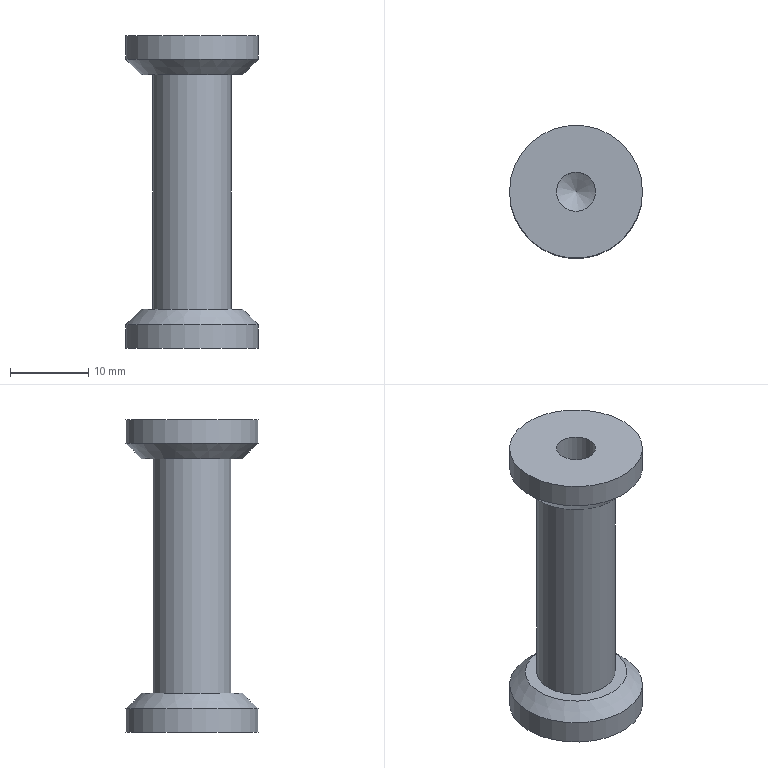Component | NX | PILLAR | 1 solid | 13 faces | box 17 x 17 x 40 mm | volume 4174 mm3 | cylinder 5 | plane 4 | cone 4 | commonest cylinder face diameters 17 x2 5 x2 10 x1
STEP:
#1=CARTESIAN_POINT('',(0.,0.,0.));
#2=DIRECTION('',(0.,0.,1.));
#3=DIRECTION('',(1.,0.,0.));
#4=AXIS2_PLACEMENT_3D('',#1,#2,#3);
#5=CARTESIAN_POINT('',(30.5,-23.75,21.));
#6=VERTEX_POINT('',#5);
#7=CARTESIAN_POINT('',(28.,-23.75,21.));
#8=DIRECTION('',(0.,0.,1.));
#9=DIRECTION('',(1.,0.,0.));
#10=AXIS2_PLACEMENT_3D('',#7,#8,#9);
#11=CIRCLE('',#10,2.5);
#12=CARTESIAN_POINT('',(28.,-32.25,21.));
#13=DIRECTION('',(0.,0.,-1.));
#14=DIRECTION('',(-1.,0.,0.));
#15=AXIS2_PLACEMENT_3D('',#12,#13,#14);
#16=PLANE('',#15);
#17=CARTESIAN_POINT('',(-2.5,8.5));
#18=CARTESIAN_POINT('',(-2.5,12.83));
#19=CARTESIAN_POINT('',(1.25,10.665));
#20=CARTESIAN_POINT('',(5.,8.5));
#21=CARTESIAN_POINT('',(1.25,6.335));
#22=CARTESIAN_POINT('',(-2.5,4.17));
#23=CARTESIAN_POINT('',(-2.5,8.5));
#24=(BOUNDED_CURVE()B_SPLINE_CURVE(2,(#17,#18,#19,#20,#21,#22,#23),.UNSPECIFIED.,.T.,.F.)B_SPLINE_CURVE_WITH_KNOTS((1,2,2,2,2,1),(-2.094,0.,2.094,4.189,6.283,8.378),.UNSPECIFIED.)CURVE()GEOMETRIC_REPRESENTATION_ITEM()RATIONAL_B_SPLINE_CURVE((1.,0.5,1.,0.5,1.,0.5,1.))REPRESENTATION_ITEM(''));
#25=(GEOMETRIC_REPRESENTATION_CONTEXT(2)PARAMETRIC_REPRESENTATION_CONTEXT()REPRESENTATION_CONTEXT('',''));
#26=DEFINITIONAL_REPRESENTATION('',(#24),#25);
#27=PCURVE('',#16,#26);
#28=CARTESIAN_POINT('',(28.,-23.75,21.));
#29=DIRECTION('',(0.,0.,1.));
#30=DIRECTION('',(1.,0.,0.));
#31=AXIS2_PLACEMENT_3D('',#28,#29,#30);
#32=CYLINDRICAL_SURFACE('',#31,2.5);
#33=CARTESIAN_POINT('',(0.,0.));
#34=DIRECTION('',(1.,0.));
#35=VECTOR('',#34,1.);
#36=LINE('',#33,#35);
#37=(GEOMETRIC_REPRESENTATION_CONTEXT(2)PARAMETRIC_REPRESENTATION_CONTEXT()REPRESENTATION_CONTEXT('',''));
#38=DEFINITIONAL_REPRESENTATION('',(#36),#37);
#39=PCURVE('',#32,#38);
#40=SURFACE_CURVE('',#11,(#27,#39),.PCURVE_S1.);
#41=EDGE_CURVE('',#6,#6,#40,.T.);
#42=ORIENTED_EDGE('',*,*,#41,.T.);
#43=EDGE_LOOP('',(#42));
#44=FACE_BOUND('',#43,.T.);
#45=CARTESIAN_POINT('',(36.5,-23.75,21.));
#46=VERTEX_POINT('',#45);
#47=CARTESIAN_POINT('',(28.,-23.75,21.));
#48=DIRECTION('',(0.,0.,1.));
#49=DIRECTION('',(1.,0.,0.));
#50=AXIS2_PLACEMENT_3D('',#47,#48,#49);
#51=CIRCLE('',#50,8.5);
#52=CARTESIAN_POINT('',(-8.5,8.5));
#53=CARTESIAN_POINT('',(-8.5,23.222));
#54=CARTESIAN_POINT('',(4.25,15.861));
#55=CARTESIAN_POINT('',(17.,8.5));
#56=CARTESIAN_POINT('',(4.25,1.139));
#57=CARTESIAN_POINT('',(-8.5,-6.222));
#58=CARTESIAN_POINT('',(-8.5,8.5));
#59=(BOUNDED_CURVE()B_SPLINE_CURVE(2,(#52,#53,#54,#55,#56,#57,#58),.UNSPECIFIED.,.T.,.F.)B_SPLINE_CURVE_WITH_KNOTS((1,2,2,2,2,1),(-2.094,0.,2.094,4.189,6.283,8.378),.UNSPECIFIED.)CURVE()GEOMETRIC_REPRESENTATION_ITEM()RATIONAL_B_SPLINE_CURVE((1.,0.5,1.,0.5,1.,0.5,1.))REPRESENTATION_ITEM(''));
#60=(GEOMETRIC_REPRESENTATION_CONTEXT(2)PARAMETRIC_REPRESENTATION_CONTEXT()REPRESENTATION_CONTEXT('',''));
#61=DEFINITIONAL_REPRESENTATION('',(#59),#60);
#62=PCURVE('',#16,#61);
#63=CARTESIAN_POINT('',(28.,-23.75,21.));
#64=DIRECTION('',(0.,0.,1.));
#65=DIRECTION('',(1.,0.,0.));
#66=AXIS2_PLACEMENT_3D('',#63,#64,#65);
#67=CYLINDRICAL_SURFACE('',#66,8.5);
#68=CARTESIAN_POINT('',(0.,0.));
#69=DIRECTION('',(1.,0.));
#70=VECTOR('',#69,1.);
#71=LINE('',#68,#70);
#72=(GEOMETRIC_REPRESENTATION_CONTEXT(2)PARAMETRIC_REPRESENTATION_CONTEXT()REPRESENTATION_CONTEXT('',''));
#73=DEFINITIONAL_REPRESENTATION('',(#71),#72);
#74=PCURVE('',#67,#73);
#75=SURFACE_CURVE('',#51,(#62,#74),.PCURVE_S1.);
#76=EDGE_CURVE('',#46,#46,#75,.T.);
#77=ORIENTED_EDGE('',*,*,#76,.F.);
#78=EDGE_LOOP('',(#77));
#79=FACE_BOUND('',#78,.T.);
#80=ADVANCED_FACE('',(#44,#79),#16,.T.);
#81=ORIENTED_EDGE('',*,*,#76,.T.);
#82=CARTESIAN_POINT('',(36.5,-23.75,24.));
#83=VERTEX_POINT('',#82);
#84=CARTESIAN_POINT('',(36.5,-23.75,21.));
#85=CARTESIAN_POINT('',(36.5,-23.75,24.));
#86=B_SPLINE_CURVE_WITH_KNOTS('',1,(#84,#85),.UNSPECIFIED.,.F.,.F.,(2,2),(0.,3.),.PIECEWISE_BEZIER_KNOTS.);
#87=CARTESIAN_POINT('',(6.283,0.));
#88=DIRECTION('',(0.,1.));
#89=VECTOR('',#88,1.);
#90=LINE('',#87,#89);
#91=(GEOMETRIC_REPRESENTATION_CONTEXT(2)PARAMETRIC_REPRESENTATION_CONTEXT()REPRESENTATION_CONTEXT('',''));
#92=DEFINITIONAL_REPRESENTATION('',(#90),#91);
#93=PCURVE('',#67,#92);
#94=CARTESIAN_POINT('',(0.,0.));
#95=DIRECTION('',(0.,1.));
#96=VECTOR('',#95,1.);
#97=LINE('',#94,#96);
#98=(GEOMETRIC_REPRESENTATION_CONTEXT(2)PARAMETRIC_REPRESENTATION_CONTEXT()REPRESENTATION_CONTEXT('',''));
#99=DEFINITIONAL_REPRESENTATION('',(#97),#98);
#100=PCURVE('',#67,#99);
#101=SEAM_CURVE('',#86,(#93,#100),.PCURVE_S1.);
#102=EDGE_CURVE('',#46,#83,#101,.T.);
#103=ORIENTED_EDGE('',*,*,#102,.T.);
#104=CARTESIAN_POINT('',(28.,-23.75,24.));
#105=DIRECTION('',(0.,0.,1.));
#106=DIRECTION('',(1.,0.,0.));
#107=AXIS2_PLACEMENT_3D('',#104,#105,#106);
#108=CIRCLE('',#107,8.5);
#109=CARTESIAN_POINT('',(0.,3.));
#110=DIRECTION('',(1.,0.));
#111=VECTOR('',#110,1.);
#112=LINE('',#109,#111);
#113=(GEOMETRIC_REPRESENTATION_CONTEXT(2)PARAMETRIC_REPRESENTATION_CONTEXT()REPRESENTATION_CONTEXT('',''));
#114=DEFINITIONAL_REPRESENTATION('',(#112),#113);
#115=PCURVE('',#67,#114);
#116=CARTESIAN_POINT('',(28.,-23.75,26.));
#117=DIRECTION('',(0.,0.,-1.));
#118=DIRECTION('',(-1.,0.,0.));
#119=AXIS2_PLACEMENT_3D('',#116,#117,#118);
#120=CONICAL_SURFACE('',#119,6.5,0.7854);
#121=CARTESIAN_POINT('',(9.425,2.));
#122=DIRECTION('',(-1.,0.));
#123=VECTOR('',#122,1.);
#124=LINE('',#121,#123);
#125=(GEOMETRIC_REPRESENTATION_CONTEXT(2)PARAMETRIC_REPRESENTATION_CONTEXT()REPRESENTATION_CONTEXT('',''));
#126=DEFINITIONAL_REPRESENTATION('',(#124),#125);
#127=PCURVE('',#120,#126);
#128=SURFACE_CURVE('',#108,(#115,#127),.PCURVE_S1.);
#129=EDGE_CURVE('',#83,#83,#128,.T.);
#130=ORIENTED_EDGE('',*,*,#129,.F.);
#131=ORIENTED_EDGE('',*,*,#102,.F.);
#132=EDGE_LOOP('',(#81,#103,#130,#131));
#133=FACE_BOUND('',#132,.T.);
#134=ADVANCED_FACE('',(#133),#67,.T.);
#135=ORIENTED_EDGE('',*,*,#129,.T.);
#136=CARTESIAN_POINT('',(34.5,-23.75,26.));
#137=VERTEX_POINT('',#136);
#138=CARTESIAN_POINT('',(34.5,-23.75,26.));
#139=CARTESIAN_POINT('',(36.5,-23.75,24.));
#140=B_SPLINE_CURVE_WITH_KNOTS('',1,(#138,#139),.UNSPECIFIED.,.F.,.F.,(2,2),(0.,2.828),.PIECEWISE_BEZIER_KNOTS.);
#141=CARTESIAN_POINT('',(3.142,0.));
#142=DIRECTION('',(0.,1.));
#143=VECTOR('',#142,1.);
#144=LINE('',#141,#143);
#145=(GEOMETRIC_REPRESENTATION_CONTEXT(2)PARAMETRIC_REPRESENTATION_CONTEXT()REPRESENTATION_CONTEXT('',''));
#146=DEFINITIONAL_REPRESENTATION('',(#144),#145);
#147=PCURVE('',#120,#146);
#148=CARTESIAN_POINT('',(9.425,0.));
#149=DIRECTION('',(0.,1.));
#150=VECTOR('',#149,1.);
#151=LINE('',#148,#150);
#152=(GEOMETRIC_REPRESENTATION_CONTEXT(2)PARAMETRIC_REPRESENTATION_CONTEXT()REPRESENTATION_CONTEXT('',''));
#153=DEFINITIONAL_REPRESENTATION('',(#151),#152);
#154=PCURVE('',#120,#153);
#155=SEAM_CURVE('',#140,(#147,#154),.PCURVE_S1.);
#156=EDGE_CURVE('',#137,#83,#155,.T.);
#157=ORIENTED_EDGE('',*,*,#156,.F.);
#158=CARTESIAN_POINT('',(28.,-23.75,26.));
#159=DIRECTION('',(0.,0.,1.));
#160=DIRECTION('',(1.,0.,0.));
#161=AXIS2_PLACEMENT_3D('',#158,#159,#160);
#162=CIRCLE('',#161,6.5);
#163=CARTESIAN_POINT('',(9.425,0.));
#164=DIRECTION('',(-1.,0.));
#165=VECTOR('',#164,1.);
#166=LINE('',#163,#165);
#167=(GEOMETRIC_REPRESENTATION_CONTEXT(2)PARAMETRIC_REPRESENTATION_CONTEXT()REPRESENTATION_CONTEXT('',''));
#168=DEFINITIONAL_REPRESENTATION('',(#166),#167);
#169=PCURVE('',#120,#168);
#170=CARTESIAN_POINT('',(28.,-28.75,26.));
#171=DIRECTION('',(0.,0.,1.));
#172=DIRECTION('',(1.,0.,0.));
#173=AXIS2_PLACEMENT_3D('',#170,#171,#172);
#174=PLANE('',#173);
#175=CARTESIAN_POINT('',(0.,5.));
#176=DIRECTION('',(1.,0.));
#177=AXIS2_PLACEMENT_2D('',#175,#176);
#178=CIRCLE('',#177,6.5);
#179=(GEOMETRIC_REPRESENTATION_CONTEXT(2)PARAMETRIC_REPRESENTATION_CONTEXT()REPRESENTATION_CONTEXT('',''));
#180=DEFINITIONAL_REPRESENTATION('',(#178),#179);
#181=PCURVE('',#174,#180);
#182=SURFACE_CURVE('',#162,(#169,#181),.PCURVE_S1.);
#183=EDGE_CURVE('',#137,#137,#182,.T.);
#184=ORIENTED_EDGE('',*,*,#183,.F.);
#185=ORIENTED_EDGE('',*,*,#156,.T.);
#186=EDGE_LOOP('',(#135,#157,#184,#185));
#187=FACE_BOUND('',#186,.T.);
#188=ADVANCED_FACE('',(#187),#120,.T.);
#189=ORIENTED_EDGE('',*,*,#183,.T.);
#190=EDGE_LOOP('',(#189));
#191=FACE_BOUND('',#190,.T.);
#192=CARTESIAN_POINT('',(33.,-23.75,26.));
#193=VERTEX_POINT('',#192);
#194=CARTESIAN_POINT('',(28.,-23.75,26.));
#195=DIRECTION('',(0.,0.,1.));
#196=DIRECTION('',(1.,0.,0.));
#197=AXIS2_PLACEMENT_3D('',#194,#195,#196);
#198=CIRCLE('',#197,5.);
#199=CARTESIAN_POINT('',(0.,5.));
#200=DIRECTION('',(1.,0.));
#201=AXIS2_PLACEMENT_2D('',#199,#200);
#202=CIRCLE('',#201,5.);
#203=(GEOMETRIC_REPRESENTATION_CONTEXT(2)PARAMETRIC_REPRESENTATION_CONTEXT()REPRESENTATION_CONTEXT('',''));
#204=DEFINITIONAL_REPRESENTATION('',(#202),#203);
#205=PCURVE('',#174,#204);
#206=CARTESIAN_POINT('',(28.,-23.75,21.));
#207=DIRECTION('',(0.,0.,1.));
#208=DIRECTION('',(1.,0.,0.));
#209=AXIS2_PLACEMENT_3D('',#206,#207,#208);
#210=CYLINDRICAL_SURFACE('',#209,5.);
#211=CARTESIAN_POINT('',(0.,5.));
#212=DIRECTION('',(1.,0.));
#213=VECTOR('',#212,1.);
#214=LINE('',#211,#213);
#215=(GEOMETRIC_REPRESENTATION_CONTEXT(2)PARAMETRIC_REPRESENTATION_CONTEXT()REPRESENTATION_CONTEXT('',''));
#216=DEFINITIONAL_REPRESENTATION('',(#214),#215);
#217=PCURVE('',#210,#216);
#218=SURFACE_CURVE('',#198,(#205,#217),.PCURVE_S1.);
#219=EDGE_CURVE('',#193,#193,#218,.T.);
#220=ORIENTED_EDGE('',*,*,#219,.F.);
#221=EDGE_LOOP('',(#220));
#222=FACE_BOUND('',#221,.T.);
#223=ADVANCED_FACE('',(#191,#222),#174,.T.);
#224=ORIENTED_EDGE('',*,*,#219,.T.);
#225=CARTESIAN_POINT('',(33.,-23.75,56.));
#226=VERTEX_POINT('',#225);
#227=CARTESIAN_POINT('',(33.,-23.75,26.));
#228=CARTESIAN_POINT('',(33.,-23.75,56.));
#229=B_SPLINE_CURVE_WITH_KNOTS('',1,(#227,#228),.UNSPECIFIED.,.F.,.F.,(2,2),(5.,35.),.PIECEWISE_BEZIER_KNOTS.);
#230=CARTESIAN_POINT('',(6.283,0.));
#231=DIRECTION('',(0.,1.));
#232=VECTOR('',#231,1.);
#233=LINE('',#230,#232);
#234=(GEOMETRIC_REPRESENTATION_CONTEXT(2)PARAMETRIC_REPRESENTATION_CONTEXT()REPRESENTATION_CONTEXT('',''));
#235=DEFINITIONAL_REPRESENTATION('',(#233),#234);
#236=PCURVE('',#210,#235);
#237=CARTESIAN_POINT('',(0.,0.));
#238=DIRECTION('',(0.,1.));
#239=VECTOR('',#238,1.);
#240=LINE('',#237,#239);
#241=(GEOMETRIC_REPRESENTATION_CONTEXT(2)PARAMETRIC_REPRESENTATION_CONTEXT()REPRESENTATION_CONTEXT('',''));
#242=DEFINITIONAL_REPRESENTATION('',(#240),#241);
#243=PCURVE('',#210,#242);
#244=SEAM_CURVE('',#229,(#236,#243),.PCURVE_S1.);
#245=EDGE_CURVE('',#193,#226,#244,.T.);
#246=ORIENTED_EDGE('',*,*,#245,.T.);
#247=CARTESIAN_POINT('',(28.,-23.75,56.));
#248=DIRECTION('',(0.,0.,1.));
#249=DIRECTION('',(1.,0.,0.));
#250=AXIS2_PLACEMENT_3D('',#247,#248,#249);
#251=CIRCLE('',#250,5.);
#252=CARTESIAN_POINT('',(0.,35.));
#253=DIRECTION('',(1.,0.));
#254=VECTOR('',#253,1.);
#255=LINE('',#252,#254);
#256=(GEOMETRIC_REPRESENTATION_CONTEXT(2)PARAMETRIC_REPRESENTATION_CONTEXT()REPRESENTATION_CONTEXT('',''));
#257=DEFINITIONAL_REPRESENTATION('',(#255),#256);
#258=PCURVE('',#210,#257);
#259=CARTESIAN_POINT('',(28.,-30.25,56.));
#260=DIRECTION('',(0.,0.,-1.));
#261=DIRECTION('',(-1.,0.,0.));
#262=AXIS2_PLACEMENT_3D('',#259,#260,#261);
#263=PLANE('',#262);
#264=CARTESIAN_POINT('',(-5.,6.5));
#265=CARTESIAN_POINT('',(-5.,15.16));
#266=CARTESIAN_POINT('',(2.5,10.83));
#267=CARTESIAN_POINT('',(10.,6.5));
#268=CARTESIAN_POINT('',(2.5,2.17));
#269=CARTESIAN_POINT('',(-5.,-2.16));
#270=CARTESIAN_POINT('',(-5.,6.5));
#271=(BOUNDED_CURVE()B_SPLINE_CURVE(2,(#264,#265,#266,#267,#268,#269,#270),.UNSPECIFIED.,.T.,.F.)B_SPLINE_CURVE_WITH_KNOTS((1,2,2,2,2,1),(-2.094,0.,2.094,4.189,6.283,8.378),.UNSPECIFIED.)CURVE()GEOMETRIC_REPRESENTATION_ITEM()RATIONAL_B_SPLINE_CURVE((1.,0.5,1.,0.5,1.,0.5,1.))REPRESENTATION_ITEM(''));
#272=(GEOMETRIC_REPRESENTATION_CONTEXT(2)PARAMETRIC_REPRESENTATION_CONTEXT()REPRESENTATION_CONTEXT('',''));
#273=DEFINITIONAL_REPRESENTATION('',(#271),#272);
#274=PCURVE('',#263,#273);
#275=SURFACE_CURVE('',#251,(#258,#274),.PCURVE_S1.);
#276=EDGE_CURVE('',#226,#226,#275,.T.);
#277=ORIENTED_EDGE('',*,*,#276,.F.);
#278=ORIENTED_EDGE('',*,*,#245,.F.);
#279=EDGE_LOOP('',(#224,#246,#277,#278));
#280=FACE_BOUND('',#279,.T.);
#281=ADVANCED_FACE('',(#280),#210,.T.);
#282=ORIENTED_EDGE('',*,*,#276,.T.);
#283=EDGE_LOOP('',(#282));
#284=FACE_BOUND('',#283,.T.);
#285=CARTESIAN_POINT('',(34.5,-23.75,56.));
#286=VERTEX_POINT('',#285);
#287=CARTESIAN_POINT('',(28.,-23.75,56.));
#288=DIRECTION('',(0.,0.,1.));
#289=DIRECTION('',(1.,0.,0.));
#290=AXIS2_PLACEMENT_3D('',#287,#288,#289);
#291=CIRCLE('',#290,6.5);
#292=CARTESIAN_POINT('',(-6.5,6.5));
#293=CARTESIAN_POINT('',(-6.5,17.758));
#294=CARTESIAN_POINT('',(3.25,12.129));
#295=CARTESIAN_POINT('',(13.,6.5));
#296=CARTESIAN_POINT('',(3.25,0.8708));
#297=CARTESIAN_POINT('',(-6.5,-4.758));
#298=CARTESIAN_POINT('',(-6.5,6.5));
#299=(BOUNDED_CURVE()B_SPLINE_CURVE(2,(#292,#293,#294,#295,#296,#297,#298),.UNSPECIFIED.,.T.,.F.)B_SPLINE_CURVE_WITH_KNOTS((1,2,2,2,2,1),(-2.094,0.,2.094,4.189,6.283,8.378),.UNSPECIFIED.)CURVE()GEOMETRIC_REPRESENTATION_ITEM()RATIONAL_B_SPLINE_CURVE((1.,0.5,1.,0.5,1.,0.5,1.))REPRESENTATION_ITEM(''));
#300=(GEOMETRIC_REPRESENTATION_CONTEXT(2)PARAMETRIC_REPRESENTATION_CONTEXT()REPRESENTATION_CONTEXT('',''));
#301=DEFINITIONAL_REPRESENTATION('',(#299),#300);
#302=PCURVE('',#263,#301);
#303=CARTESIAN_POINT('',(28.,-23.75,58.));
#304=DIRECTION('',(0.,0.,1.));
#305=DIRECTION('',(1.,0.,0.));
#306=AXIS2_PLACEMENT_3D('',#303,#304,#305);
#307=CONICAL_SURFACE('',#306,8.5,0.7854);
#308=CARTESIAN_POINT('',(0.,-2.));
#309=DIRECTION('',(1.,0.));
#310=VECTOR('',#309,1.);
#311=LINE('',#308,#310);
#312=(GEOMETRIC_REPRESENTATION_CONTEXT(2)PARAMETRIC_REPRESENTATION_CONTEXT()REPRESENTATION_CONTEXT('',''));
#313=DEFINITIONAL_REPRESENTATION('',(#311),#312);
#314=PCURVE('',#307,#313);
#315=SURFACE_CURVE('',#291,(#302,#314),.PCURVE_S1.);
#316=EDGE_CURVE('',#286,#286,#315,.T.);
#317=ORIENTED_EDGE('',*,*,#316,.F.);
#318=EDGE_LOOP('',(#317));
#319=FACE_BOUND('',#318,.T.);
#320=ADVANCED_FACE('',(#284,#319),#263,.T.);
#321=ORIENTED_EDGE('',*,*,#316,.T.);
#322=CARTESIAN_POINT('',(36.5,-23.75,58.));
#323=VERTEX_POINT('',#322);
#324=CARTESIAN_POINT('',(34.5,-23.75,56.));
#325=CARTESIAN_POINT('',(36.5,-23.75,58.));
#326=B_SPLINE_CURVE_WITH_KNOTS('',1,(#324,#325),.UNSPECIFIED.,.F.,.F.,(2,2),(-2.828,0.),.PIECEWISE_BEZIER_KNOTS.);
#327=CARTESIAN_POINT('',(6.283,0.));
#328=DIRECTION('',(0.,1.));
#329=VECTOR('',#328,1.);
#330=LINE('',#327,#329);
#331=(GEOMETRIC_REPRESENTATION_CONTEXT(2)PARAMETRIC_REPRESENTATION_CONTEXT()REPRESENTATION_CONTEXT('',''));
#332=DEFINITIONAL_REPRESENTATION('',(#330),#331);
#333=PCURVE('',#307,#332);
#334=CARTESIAN_POINT('',(0.,0.));
#335=DIRECTION('',(0.,1.));
#336=VECTOR('',#335,1.);
#337=LINE('',#334,#336);
#338=(GEOMETRIC_REPRESENTATION_CONTEXT(2)PARAMETRIC_REPRESENTATION_CONTEXT()REPRESENTATION_CONTEXT('',''));
#339=DEFINITIONAL_REPRESENTATION('',(#337),#338);
#340=PCURVE('',#307,#339);
#341=SEAM_CURVE('',#326,(#333,#340),.PCURVE_S1.);
#342=EDGE_CURVE('',#286,#323,#341,.T.);
#343=ORIENTED_EDGE('',*,*,#342,.T.);
#344=CARTESIAN_POINT('',(28.,-23.75,58.));
#345=DIRECTION('',(0.,0.,1.));
#346=DIRECTION('',(1.,0.,0.));
#347=AXIS2_PLACEMENT_3D('',#344,#345,#346);
#348=CIRCLE('',#347,8.5);
#349=CARTESIAN_POINT('',(0.,0.));
#350=DIRECTION('',(1.,0.));
#351=VECTOR('',#350,1.);
#352=LINE('',#349,#351);
#353=(GEOMETRIC_REPRESENTATION_CONTEXT(2)PARAMETRIC_REPRESENTATION_CONTEXT()REPRESENTATION_CONTEXT('',''));
#354=DEFINITIONAL_REPRESENTATION('',(#352),#353);
#355=PCURVE('',#307,#354);
#356=CARTESIAN_POINT('',(28.,-23.75,21.));
#357=DIRECTION('',(0.,0.,1.));
#358=DIRECTION('',(1.,0.,0.));
#359=AXIS2_PLACEMENT_3D('',#356,#357,#358);
#360=CYLINDRICAL_SURFACE('',#359,8.5);
#361=CARTESIAN_POINT('',(0.,37.));
#362=DIRECTION('',(1.,0.));
#363=VECTOR('',#362,1.);
#364=LINE('',#361,#363);
#365=(GEOMETRIC_REPRESENTATION_CONTEXT(2)PARAMETRIC_REPRESENTATION_CONTEXT()REPRESENTATION_CONTEXT('',''));
#366=DEFINITIONAL_REPRESENTATION('',(#364),#365);
#367=PCURVE('',#360,#366);
#368=SURFACE_CURVE('',#348,(#355,#367),.PCURVE_S1.);
#369=EDGE_CURVE('',#323,#323,#368,.T.);
#370=ORIENTED_EDGE('',*,*,#369,.F.);
#371=ORIENTED_EDGE('',*,*,#342,.F.);
#372=EDGE_LOOP('',(#321,#343,#370,#371));
#373=FACE_BOUND('',#372,.T.);
#374=ADVANCED_FACE('',(#373),#307,.T.);
#375=ORIENTED_EDGE('',*,*,#369,.T.);
#376=CARTESIAN_POINT('',(36.5,-23.75,61.));
#377=VERTEX_POINT('',#376);
#378=CARTESIAN_POINT('',(36.5,-23.75,58.));
#379=CARTESIAN_POINT('',(36.5,-23.75,61.));
#380=B_SPLINE_CURVE_WITH_KNOTS('',1,(#378,#379),.UNSPECIFIED.,.F.,.F.,(2,2),(37.,40.),.PIECEWISE_BEZIER_KNOTS.);
#381=CARTESIAN_POINT('',(6.283,0.));
#382=DIRECTION('',(0.,1.));
#383=VECTOR('',#382,1.);
#384=LINE('',#381,#383);
#385=(GEOMETRIC_REPRESENTATION_CONTEXT(2)PARAMETRIC_REPRESENTATION_CONTEXT()REPRESENTATION_CONTEXT('',''));
#386=DEFINITIONAL_REPRESENTATION('',(#384),#385);
#387=PCURVE('',#360,#386);
#388=CARTESIAN_POINT('',(0.,0.));
#389=DIRECTION('',(0.,1.));
#390=VECTOR('',#389,1.);
#391=LINE('',#388,#390);
#392=(GEOMETRIC_REPRESENTATION_CONTEXT(2)PARAMETRIC_REPRESENTATION_CONTEXT()REPRESENTATION_CONTEXT('',''));
#393=DEFINITIONAL_REPRESENTATION('',(#391),#392);
#394=PCURVE('',#360,#393);
#395=SEAM_CURVE('',#380,(#387,#394),.PCURVE_S1.);
#396=EDGE_CURVE('',#323,#377,#395,.T.);
#397=ORIENTED_EDGE('',*,*,#396,.T.);
#398=CARTESIAN_POINT('',(28.,-23.75,61.));
#399=DIRECTION('',(0.,0.,1.));
#400=DIRECTION('',(1.,0.,0.));
#401=AXIS2_PLACEMENT_3D('',#398,#399,#400);
#402=CIRCLE('',#401,8.5);
#403=CARTESIAN_POINT('',(0.,40.));
#404=DIRECTION('',(1.,0.));
#405=VECTOR('',#404,1.);
#406=LINE('',#403,#405);
#407=(GEOMETRIC_REPRESENTATION_CONTEXT(2)PARAMETRIC_REPRESENTATION_CONTEXT()REPRESENTATION_CONTEXT('',''));
#408=DEFINITIONAL_REPRESENTATION('',(#406),#407);
#409=PCURVE('',#360,#408);
#410=CARTESIAN_POINT('',(28.,-23.75,61.));
#411=DIRECTION('',(0.,0.,1.));
#412=DIRECTION('',(1.,0.,0.));
#413=AXIS2_PLACEMENT_3D('',#410,#411,#412);
#414=PLANE('',#413);
#415=CARTESIAN_POINT('',(0.,0.));
#416=DIRECTION('',(1.,0.));
#417=AXIS2_PLACEMENT_2D('',#415,#416);
#418=CIRCLE('',#417,8.5);
#419=(GEOMETRIC_REPRESENTATION_CONTEXT(2)PARAMETRIC_REPRESENTATION_CONTEXT()REPRESENTATION_CONTEXT('',''));
#420=DEFINITIONAL_REPRESENTATION('',(#418),#419);
#421=PCURVE('',#414,#420);
#422=SURFACE_CURVE('',#402,(#409,#421),.PCURVE_S1.);
#423=EDGE_CURVE('',#377,#377,#422,.T.);
#424=ORIENTED_EDGE('',*,*,#423,.F.);
#425=ORIENTED_EDGE('',*,*,#396,.F.);
#426=EDGE_LOOP('',(#375,#397,#424,#425));
#427=FACE_BOUND('',#426,.T.);
#428=ADVANCED_FACE('',(#427),#360,.T.);
#429=CARTESIAN_POINT('',(25.5,-23.75,61.));
#430=VERTEX_POINT('',#429);
#431=CARTESIAN_POINT('',(28.,-23.75,61.));
#432=DIRECTION('',(0.,0.,-1.));
#433=DIRECTION('',(-1.,0.,0.));
#434=AXIS2_PLACEMENT_3D('',#431,#432,#433);
#435=CIRCLE('',#434,2.5);
#436=CARTESIAN_POINT('',(-2.5,0.));
#437=CARTESIAN_POINT('',(-2.5,4.33));
#438=CARTESIAN_POINT('',(1.25,2.165));
#439=CARTESIAN_POINT('',(5.,0.));
#440=CARTESIAN_POINT('',(1.25,-2.165));
#441=CARTESIAN_POINT('',(-2.5,-4.33));
#442=CARTESIAN_POINT('',(-2.5,0.));
#443=(BOUNDED_CURVE()B_SPLINE_CURVE(2,(#436,#437,#438,#439,#440,#441,#442),.UNSPECIFIED.,.T.,.F.)B_SPLINE_CURVE_WITH_KNOTS((1,2,2,2,2,1),(-2.094,0.,2.094,4.189,6.283,8.378),.UNSPECIFIED.)CURVE()GEOMETRIC_REPRESENTATION_ITEM()RATIONAL_B_SPLINE_CURVE((1.,0.5,1.,0.5,1.,0.5,1.))REPRESENTATION_ITEM(''));
#444=(GEOMETRIC_REPRESENTATION_CONTEXT(2)PARAMETRIC_REPRESENTATION_CONTEXT()REPRESENTATION_CONTEXT('',''));
#445=DEFINITIONAL_REPRESENTATION('',(#443),#444);
#446=PCURVE('',#414,#445);
#447=CARTESIAN_POINT('',(28.,-23.75,61.));
#448=DIRECTION('',(0.,0.,-1.));
#449=DIRECTION('',(-1.,0.,0.));
#450=AXIS2_PLACEMENT_3D('',#447,#448,#449);
#451=CYLINDRICAL_SURFACE('',#450,2.5);
#452=CARTESIAN_POINT('',(0.,0.));
#453=DIRECTION('',(1.,0.));
#454=VECTOR('',#453,1.);
#455=LINE('',#452,#454);
#456=(GEOMETRIC_REPRESENTATION_CONTEXT(2)PARAMETRIC_REPRESENTATION_CONTEXT()REPRESENTATION_CONTEXT('',''));
#457=DEFINITIONAL_REPRESENTATION('',(#455),#456);
#458=PCURVE('',#451,#457);
#459=SURFACE_CURVE('',#435,(#446,#458),.PCURVE_S1.);
#460=EDGE_CURVE('',#430,#430,#459,.T.);
#461=ORIENTED_EDGE('',*,*,#460,.T.);
#462=EDGE_LOOP('',(#461));
#463=FACE_BOUND('',#462,.T.);
#464=ORIENTED_EDGE('',*,*,#423,.T.);
#465=EDGE_LOOP('',(#464));
#466=FACE_BOUND('',#465,.T.);
#467=ADVANCED_FACE('',(#463,#466),#414,.T.);
#468=CARTESIAN_POINT('',(30.5,-23.75,55.));
#469=VERTEX_POINT('',#468);
#470=CARTESIAN_POINT('',(25.5,-23.75,55.));
#471=VERTEX_POINT('',#470);
#472=CARTESIAN_POINT('',(28.,-23.75,55.));
#473=DIRECTION('',(0.,0.,1.));
#474=DIRECTION('',(-1.,0.,0.));
#475=AXIS2_PLACEMENT_3D('',#472,#473,#474);
#476=CIRCLE('',#475,2.5);
#477=CARTESIAN_POINT('',(28.,-23.75,55.));
#478=DIRECTION('',(0.,0.,1.));
#479=DIRECTION('',(1.,0.,0.));
#480=AXIS2_PLACEMENT_3D('',#477,#478,#479);
#481=CONICAL_SURFACE('',#480,2.5,1.03);
#482=CARTESIAN_POINT('',(-3.142,0.));
#483=DIRECTION('',(1.,0.));
#484=VECTOR('',#483,1.);
#485=LINE('',#482,#484);
#486=(GEOMETRIC_REPRESENTATION_CONTEXT(2)PARAMETRIC_REPRESENTATION_CONTEXT()REPRESENTATION_CONTEXT('',''));
#487=DEFINITIONAL_REPRESENTATION('',(#485),#486);
#488=PCURVE('',#481,#487);
#489=CARTESIAN_POINT('',(6.283,6.));
#490=DIRECTION('',(-1.,0.));
#491=VECTOR('',#490,1.);
#492=LINE('',#489,#491);
#493=(GEOMETRIC_REPRESENTATION_CONTEXT(2)PARAMETRIC_REPRESENTATION_CONTEXT()REPRESENTATION_CONTEXT('',''));
#494=DEFINITIONAL_REPRESENTATION('',(#492),#493);
#495=PCURVE('',#451,#494);
#496=SURFACE_CURVE('',#476,(#488,#495),.PCURVE_S1.);
#497=EDGE_CURVE('',#469,#471,#496,.T.);
#498=ORIENTED_EDGE('',*,*,#497,.F.);
#499=CARTESIAN_POINT('',(28.,-23.75,53.498));
#500=VERTEX_POINT('',#499);
#501=CARTESIAN_POINT('',(28.,-23.75,53.498));
#502=CARTESIAN_POINT('',(30.5,-23.75,55.));
#503=B_SPLINE_CURVE_WITH_KNOTS('',1,(#501,#502),.UNSPECIFIED.,.F.,.F.,(2,2),(-2.917,0.),.PIECEWISE_BEZIER_KNOTS.);
#504=CARTESIAN_POINT('',(0.,0.));
#505=DIRECTION('',(0.,1.));
#506=VECTOR('',#505,1.);
#507=LINE('',#504,#506);
#508=(GEOMETRIC_REPRESENTATION_CONTEXT(2)PARAMETRIC_REPRESENTATION_CONTEXT()REPRESENTATION_CONTEXT('',''));
#509=DEFINITIONAL_REPRESENTATION('',(#507),#508);
#510=PCURVE('',#481,#509);
#511=CARTESIAN_POINT('',(6.283,0.));
#512=DIRECTION('',(0.,1.));
#513=VECTOR('',#512,1.);
#514=LINE('',#511,#513);
#515=(GEOMETRIC_REPRESENTATION_CONTEXT(2)PARAMETRIC_REPRESENTATION_CONTEXT()REPRESENTATION_CONTEXT('',''));
#516=DEFINITIONAL_REPRESENTATION('',(#514),#515);
#517=PCURVE('',#481,#516);
#518=SEAM_CURVE('',#503,(#510,#517),.PCURVE_S1.);
#519=EDGE_CURVE('',#500,#469,#518,.T.);
#520=ORIENTED_EDGE('',*,*,#519,.F.);
#521=ORIENTED_EDGE('',*,*,#519,.T.);
#522=CARTESIAN_POINT('',(28.,-23.75,55.));
#523=DIRECTION('',(0.,0.,1.));
#524=DIRECTION('',(-1.,0.,0.));
#525=AXIS2_PLACEMENT_3D('',#522,#523,#524);
#526=CIRCLE('',#525,2.5);
#527=CARTESIAN_POINT('',(3.142,0.));
#528=DIRECTION('',(1.,0.));
#529=VECTOR('',#528,1.);
#530=LINE('',#527,#529);
#531=(GEOMETRIC_REPRESENTATION_CONTEXT(2)PARAMETRIC_REPRESENTATION_CONTEXT()REPRESENTATION_CONTEXT('',''));
#532=DEFINITIONAL_REPRESENTATION('',(#530),#531);
#533=PCURVE('',#481,#532);
#534=CARTESIAN_POINT('',(6.283,6.));
#535=DIRECTION('',(-1.,0.));
#536=VECTOR('',#535,1.);
#537=LINE('',#534,#536);
#538=(GEOMETRIC_REPRESENTATION_CONTEXT(2)PARAMETRIC_REPRESENTATION_CONTEXT()REPRESENTATION_CONTEXT('',''));
#539=DEFINITIONAL_REPRESENTATION('',(#537),#538);
#540=PCURVE('',#451,#539);
#541=SURFACE_CURVE('',#526,(#533,#540),.PCURVE_S1.);
#542=EDGE_CURVE('',#471,#469,#541,.T.);
#543=ORIENTED_EDGE('',*,*,#542,.F.);
#544=EDGE_LOOP('',(#498,#520,#521,#543));
#545=FACE_BOUND('',#544,.F.);
#546=ADVANCED_FACE('',(#545),#481,.F.);
#547=ORIENTED_EDGE('',*,*,#497,.T.);
#548=CARTESIAN_POINT('',(25.5,-23.75,61.));
#549=CARTESIAN_POINT('',(25.5,-23.75,55.));
#550=B_SPLINE_CURVE_WITH_KNOTS('',1,(#548,#549),.UNSPECIFIED.,.F.,.F.,(2,2),(0.,6.),.PIECEWISE_BEZIER_KNOTS.);
#551=CARTESIAN_POINT('',(0.,0.));
#552=DIRECTION('',(0.,1.));
#553=VECTOR('',#552,1.);
#554=LINE('',#551,#553);
#555=(GEOMETRIC_REPRESENTATION_CONTEXT(2)PARAMETRIC_REPRESENTATION_CONTEXT()REPRESENTATION_CONTEXT('',''));
#556=DEFINITIONAL_REPRESENTATION('',(#554),#555);
#557=PCURVE('',#451,#556);
#558=CARTESIAN_POINT('',(6.283,0.));
#559=DIRECTION('',(0.,1.));
#560=VECTOR('',#559,1.);
#561=LINE('',#558,#560);
#562=(GEOMETRIC_REPRESENTATION_CONTEXT(2)PARAMETRIC_REPRESENTATION_CONTEXT()REPRESENTATION_CONTEXT('',''));
#563=DEFINITIONAL_REPRESENTATION('',(#561),#562);
#564=PCURVE('',#451,#563);
#565=SEAM_CURVE('',#550,(#557,#564),.PCURVE_S1.);
#566=EDGE_CURVE('',#430,#471,#565,.T.);
#567=ORIENTED_EDGE('',*,*,#566,.F.);
#568=ORIENTED_EDGE('',*,*,#460,.T.);
#569=ORIENTED_EDGE('',*,*,#566,.T.);
#570=ORIENTED_EDGE('',*,*,#542,.T.);
#571=EDGE_LOOP('',(#547,#567,#568,#569,#570));
#572=FACE_BOUND('',#571,.F.);
#573=ADVANCED_FACE('',(#572),#451,.F.);
#574=CARTESIAN_POINT('',(25.5,-23.75,27.));
#575=VERTEX_POINT('',#574);
#576=CARTESIAN_POINT('',(30.5,-23.75,27.));
#577=VERTEX_POINT('',#576);
#578=CARTESIAN_POINT('',(28.,-23.75,27.));
#579=DIRECTION('',(0.,0.,-1.));
#580=DIRECTION('',(1.,0.,0.));
#581=AXIS2_PLACEMENT_3D('',#578,#579,#580);
#582=CIRCLE('',#581,2.5);
#583=CARTESIAN_POINT('',(28.,-23.75,27.));
#584=DIRECTION('',(0.,0.,-1.));
#585=DIRECTION('',(-1.,0.,0.));
#586=AXIS2_PLACEMENT_3D('',#583,#584,#585);
#587=CONICAL_SURFACE('',#586,2.5,1.03);
#588=CARTESIAN_POINT('',(-3.142,0.));
#589=DIRECTION('',(1.,0.));
#590=VECTOR('',#589,1.);
#591=LINE('',#588,#590);
#592=(GEOMETRIC_REPRESENTATION_CONTEXT(2)PARAMETRIC_REPRESENTATION_CONTEXT()REPRESENTATION_CONTEXT('',''));
#593=DEFINITIONAL_REPRESENTATION('',(#591),#592);
#594=PCURVE('',#587,#593);
#595=CARTESIAN_POINT('',(6.283,6.));
#596=DIRECTION('',(-1.,0.));
#597=VECTOR('',#596,1.);
#598=LINE('',#595,#597);
#599=(GEOMETRIC_REPRESENTATION_CONTEXT(2)PARAMETRIC_REPRESENTATION_CONTEXT()REPRESENTATION_CONTEXT('',''));
#600=DEFINITIONAL_REPRESENTATION('',(#598),#599);
#601=PCURVE('',#32,#600);
#602=SURFACE_CURVE('',#582,(#594,#601),.PCURVE_S1.);
#603=EDGE_CURVE('',#575,#577,#602,.T.);
#604=ORIENTED_EDGE('',*,*,#603,.F.);
#605=CARTESIAN_POINT('',(28.,-23.75,28.502));
#606=VERTEX_POINT('',#605);
#607=CARTESIAN_POINT('',(28.,-23.75,28.502));
#608=CARTESIAN_POINT('',(25.5,-23.75,27.));
#609=B_SPLINE_CURVE_WITH_KNOTS('',1,(#607,#608),.UNSPECIFIED.,.F.,.F.,(2,2),(-2.917,0.),.PIECEWISE_BEZIER_KNOTS.);
#610=CARTESIAN_POINT('',(0.,0.));
#611=DIRECTION('',(0.,1.));
#612=VECTOR('',#611,1.);
#613=LINE('',#610,#612);
#614=(GEOMETRIC_REPRESENTATION_CONTEXT(2)PARAMETRIC_REPRESENTATION_CONTEXT()REPRESENTATION_CONTEXT('',''));
#615=DEFINITIONAL_REPRESENTATION('',(#613),#614);
#616=PCURVE('',#587,#615);
#617=CARTESIAN_POINT('',(6.283,0.));
#618=DIRECTION('',(0.,1.));
#619=VECTOR('',#618,1.);
#620=LINE('',#617,#619);
#621=(GEOMETRIC_REPRESENTATION_CONTEXT(2)PARAMETRIC_REPRESENTATION_CONTEXT()REPRESENTATION_CONTEXT('',''));
#622=DEFINITIONAL_REPRESENTATION('',(#620),#621);
#623=PCURVE('',#587,#622);
#624=SEAM_CURVE('',#609,(#616,#623),.PCURVE_S1.);
#625=EDGE_CURVE('',#606,#575,#624,.T.);
#626=ORIENTED_EDGE('',*,*,#625,.F.);
#627=ORIENTED_EDGE('',*,*,#625,.T.);
#628=CARTESIAN_POINT('',(28.,-23.75,27.));
#629=DIRECTION('',(0.,0.,-1.));
#630=DIRECTION('',(1.,0.,0.));
#631=AXIS2_PLACEMENT_3D('',#628,#629,#630);
#632=CIRCLE('',#631,2.5);
#633=CARTESIAN_POINT('',(3.142,0.));
#634=DIRECTION('',(1.,0.));
#635=VECTOR('',#634,1.);
#636=LINE('',#633,#635);
#637=(GEOMETRIC_REPRESENTATION_CONTEXT(2)PARAMETRIC_REPRESENTATION_CONTEXT()REPRESENTATION_CONTEXT('',''));
#638=DEFINITIONAL_REPRESENTATION('',(#636),#637);
#639=PCURVE('',#587,#638);
#640=CARTESIAN_POINT('',(6.283,6.));
#641=DIRECTION('',(-1.,0.));
#642=VECTOR('',#641,1.);
#643=LINE('',#640,#642);
#644=(GEOMETRIC_REPRESENTATION_CONTEXT(2)PARAMETRIC_REPRESENTATION_CONTEXT()REPRESENTATION_CONTEXT('',''));
#645=DEFINITIONAL_REPRESENTATION('',(#643),#644);
#646=PCURVE('',#32,#645);
#647=SURFACE_CURVE('',#632,(#639,#646),.PCURVE_S1.);
#648=EDGE_CURVE('',#577,#575,#647,.T.);
#649=ORIENTED_EDGE('',*,*,#648,.F.);
#650=EDGE_LOOP('',(#604,#626,#627,#649));
#651=FACE_BOUND('',#650,.F.);
#652=ADVANCED_FACE('',(#651),#587,.F.);
#653=ORIENTED_EDGE('',*,*,#603,.T.);
#654=CARTESIAN_POINT('',(30.5,-23.75,21.));
#655=CARTESIAN_POINT('',(30.5,-23.75,27.));
#656=B_SPLINE_CURVE_WITH_KNOTS('',1,(#654,#655),.UNSPECIFIED.,.F.,.F.,(2,2),(0.,6.),.PIECEWISE_BEZIER_KNOTS.);
#657=CARTESIAN_POINT('',(0.,0.));
#658=DIRECTION('',(0.,1.));
#659=VECTOR('',#658,1.);
#660=LINE('',#657,#659);
#661=(GEOMETRIC_REPRESENTATION_CONTEXT(2)PARAMETRIC_REPRESENTATION_CONTEXT()REPRESENTATION_CONTEXT('',''));
#662=DEFINITIONAL_REPRESENTATION('',(#660),#661);
#663=PCURVE('',#32,#662);
#664=CARTESIAN_POINT('',(6.283,0.));
#665=DIRECTION('',(0.,1.));
#666=VECTOR('',#665,1.);
#667=LINE('',#664,#666);
#668=(GEOMETRIC_REPRESENTATION_CONTEXT(2)PARAMETRIC_REPRESENTATION_CONTEXT()REPRESENTATION_CONTEXT('',''));
#669=DEFINITIONAL_REPRESENTATION('',(#667),#668);
#670=PCURVE('',#32,#669);
#671=SEAM_CURVE('',#656,(#663,#670),.PCURVE_S1.);
#672=EDGE_CURVE('',#6,#577,#671,.T.);
#673=ORIENTED_EDGE('',*,*,#672,.F.);
#674=ORIENTED_EDGE('',*,*,#41,.T.);
#675=ORIENTED_EDGE('',*,*,#672,.T.);
#676=ORIENTED_EDGE('',*,*,#648,.T.);
#677=EDGE_LOOP('',(#653,#673,#674,#675,#676));
#678=FACE_BOUND('',#677,.F.);
#679=ADVANCED_FACE('',(#678),#32,.F.);
#680=CLOSED_SHELL('',(#80,#134,#188,#223,#281,#320,#374,#428,#467,#546,#573,#652,#679));
#681=MANIFOLD_SOLID_BREP('',#680);
#682=(LENGTH_UNIT()NAMED_UNIT(*)SI_UNIT(.MILLI.,.METRE.));
#683=UNCERTAINTY_MEASURE_WITH_UNIT(LENGTH_MEASURE(0.00001),#682,'','');
#684=(NAMED_UNIT(*)PLANE_ANGLE_UNIT()SI_UNIT($,.RADIAN.));
#685=(NAMED_UNIT(*)SI_UNIT($,.STERADIAN.)SOLID_ANGLE_UNIT());
#686=(GEOMETRIC_REPRESENTATION_CONTEXT(3)GLOBAL_UNCERTAINTY_ASSIGNED_CONTEXT((#683))GLOBAL_UNIT_ASSIGNED_CONTEXT((#682,#684,#685))REPRESENTATION_CONTEXT('',''));
#687=ADVANCED_BREP_SHAPE_REPRESENTATION('',(#4,#681),#686);